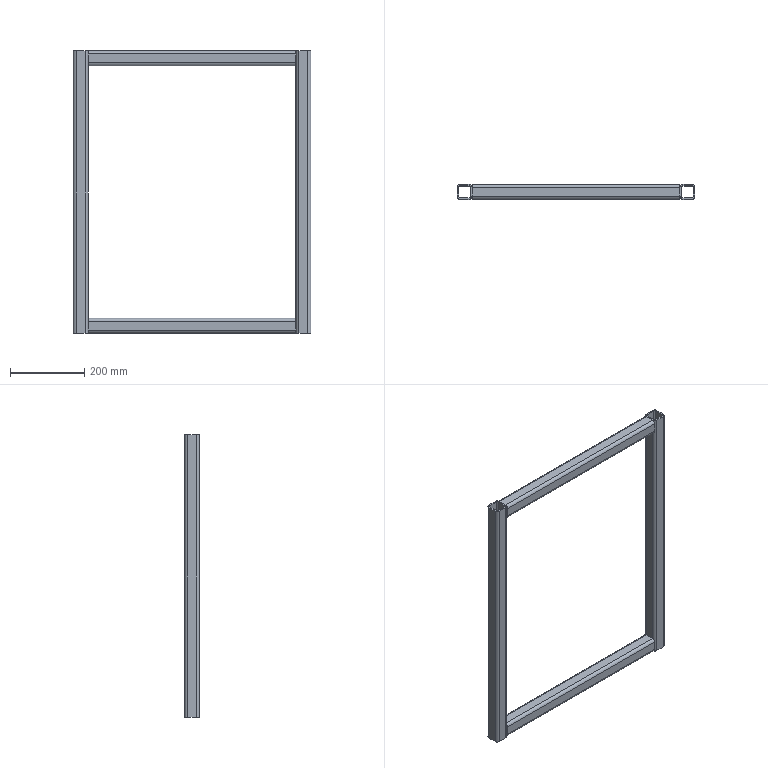Component | SolidWorks | 01-01Chassis-1_01-01-01ChassisWeldment1-1 | 4 solids | 74 faces | box 640 x 40 x 760 mm | volume 1411290 mm3 | plane 40 | cylinder 34 | commonest cylinder face diameters 8 x16 16 x16 13.5 x2 | material Q235
build123d program:
from build123d import *

# Parameters (mm, degrees)
SQUARE_TUBE_40_X_40_X_4_1_DEPTH   = 600
SQUARE_TUBE_40_X_40_X_4_1_2_DEPTH = 600
SQUARE_TUBE_40_X_40_X_4_2_DEPTH   = 720
SQUARE_TUBE_40_X_40_X_4_2_2_DEPTH = 720
BODY_3_RUN_ON_DEPTH               = 20
BODY_START                        = 720
BODY_3_RUN_ON_2_DEPTH             = 20
BODY_4_RUN_ON_DEPTH               = 20
BODY_4_RUN_ON_2_DEPTH             = 20
SKETCH13_R                        = 6.75
CUT_EXTRUDE1_DEPTH                = 10


with BuildPart() as part:
    # Sketch12 → Square Tube 40 X 40 X 4_1 (new body)
    with BuildSketch(Plane(origin=(300, 0, -360), x_dir=(0, 0, 1), z_dir=(-1, 0, 0))):
        with BuildLine():
            Line((-12, -20), (12, -20))
            ThreePointArc((12, -20), (17.657, -17.657), (20, -12))
            Line((20, -12), (20, 12))
            ThreePointArc((20, 12), (17.657, 17.657), (12, 20))
            Line((12, 20), (-12, 20))
            ThreePointArc((-12, 20), (-17.657, 17.657), (-20, 12))
            Line((-20, 12), (-20, -12))
            ThreePointArc((-20, -12), (-17.657, -17.657), (-12, -20))
        make_face()
        with BuildLine():
            Line((-12, -16), (12, -16))
            ThreePointArc((12, -16), (14.828, -14.828), (16, -12))
            Line((16, -12), (16, 12))
            ThreePointArc((16, 12), (14.828, 14.828), (12, 16))
            Line((12, 16), (-12, 16))
            ThreePointArc((-12, 16), (-14.828, 14.828), (-16, 12))
            Line((-16, 12), (-16, -12))
            ThreePointArc((-16, -12), (-14.828, -14.828), (-12, -16))
        make_face(mode=Mode.SUBTRACT)
    extrude(amount=SQUARE_TUBE_40_X_40_X_4_1_DEPTH)

    # Trim_Extend2 12
    split(bisect_by=Plane(origin=(-284, 0, 10), x_dir=(0, 1, 0), z_dir=(1, 0, 0)), keep=Keep.TOP)

    # Trim_Extend2 15
    split(bisect_by=Plane(origin=(-280, 0, 10), x_dir=(0, 1, 0), z_dir=(1, 0, 0)), keep=Keep.TOP)

    # Trim_Extend4 9
    split(bisect_by=Plane(origin=(280, 0, 0), x_dir=(0, -1, 0), z_dir=(-1, 0, 0)), keep=Keep.TOP)


with BuildPart() as body_2:
    # Sketch12 on segment 2 (on carried to segment 2) → Square Tube 40 X 40 X 4_1 2 (new body)
    with BuildSketch(Plane(origin=(300, 0, 360), x_dir=(0, 0, 1), z_dir=(-1, 0, 0))):
        with BuildLine():
            Line((-12, -20), (12, -20))
            ThreePointArc((12, -20), (17.657, -17.657), (20, -12))
            Line((20, -12), (20, 12))
            ThreePointArc((20, 12), (17.657, 17.657), (12, 20))
            Line((12, 20), (-12, 20))
            ThreePointArc((-12, 20), (-17.657, 17.657), (-20, 12))
            Line((-20, 12), (-20, -12))
            ThreePointArc((-20, -12), (-17.657, -17.657), (-12, -20))
        make_face()
        with BuildLine():
            Line((-12, -16), (12, -16))
            ThreePointArc((12, -16), (14.828, -14.828), (16, -12))
            Line((16, -12), (16, 12))
            ThreePointArc((16, 12), (14.828, 14.828), (12, 16))
            Line((12, 16), (-12, 16))
            ThreePointArc((-12, 16), (-14.828, 14.828), (-16, 12))
            Line((-16, 12), (-16, -12))
            ThreePointArc((-16, -12), (-14.828, -14.828), (-12, -16))
        make_face(mode=Mode.SUBTRACT)
    extrude(amount=SQUARE_TUBE_40_X_40_X_4_1_2_DEPTH)

    # Trim_Extend1 11
    split(bisect_by=Plane.YZ.offset(-280), keep=Keep.TOP)

    # Trim_Extend6 10
    split(bisect_by=Plane(origin=(284, 0, -10), x_dir=(0, -1, 0), z_dir=(-1, 0, 0)), keep=Keep.TOP)

    # Trim_Extend6 13
    split(bisect_by=Plane(origin=(280, 0, -10), x_dir=(0, -1, 0), z_dir=(-1, 0, 0)), keep=Keep.TOP)


with BuildPart() as body_3:
    # Sketch1 → Square Tube 40 X 40 X 4_2 (new body)
    with BuildSketch(Plane(origin=(-300, 0, 360), x_dir=(-1, 0, 0), z_dir=(0, 0, -1))):
        with BuildLine():
            Line((-12, -20), (12, -20))
            ThreePointArc((12, -20), (17.657, -17.657), (20, -12))
            Line((20, -12), (20, 12))
            ThreePointArc((20, 12), (17.657, 17.657), (12, 20))
            Line((12, 20), (-12, 20))
            ThreePointArc((-12, 20), (-17.657, 17.657), (-20, 12))
            Line((-20, 12), (-20, -12))
            ThreePointArc((-20, -12), (-17.657, -17.657), (-12, -20))
        make_face()
        with BuildLine():
            Line((-12, -16), (12, -16))
            ThreePointArc((12, -16), (14.828, -14.828), (16, -12))
            Line((16, -12), (16, 12))
            ThreePointArc((16, 12), (14.828, 14.828), (12, 16))
            Line((12, 16), (-12, 16))
            ThreePointArc((-12, 16), (-14.828, 14.828), (-16, 12))
            Line((-16, 12), (-16, -12))
            ThreePointArc((-16, -12), (-14.828, -14.828), (-12, -16))
        make_face(mode=Mode.SUBTRACT)
    extrude(amount=SQUARE_TUBE_40_X_40_X_4_2_DEPTH)

    # Sketch1 → body 3 run on (add)
    with BuildSketch(Plane(origin=(-300, 0, 360), x_dir=(-1, 0, 0), z_dir=(0, 0, -1))):
        with BuildLine():
            Line((-12, -20), (12, -20))
            ThreePointArc((12, -20), (17.657, -17.657), (20, -12))
            Line((20, -12), (20, 12))
            ThreePointArc((20, 12), (17.657, 17.657), (12, 20))
            Line((12, 20), (-12, 20))
            ThreePointArc((-12, 20), (-17.657, 17.657), (-20, 12))
            Line((-20, 12), (-20, -12))
            ThreePointArc((-20, -12), (-17.657, -17.657), (-12, -20))
        make_face()
        with BuildLine():
            Line((-12, -16), (12, -16))
            ThreePointArc((12, -16), (14.828, -14.828), (16, -12))
            Line((16, -12), (16, 12))
            ThreePointArc((16, 12), (14.828, 14.828), (12, 16))
            Line((12, 16), (-12, 16))
            ThreePointArc((-12, 16), (-14.828, 14.828), (-16, 12))
            Line((-16, 12), (-16, -12))
            ThreePointArc((-16, -12), (-14.828, -14.828), (-12, -16))
        make_face(mode=Mode.SUBTRACT)
    extrude(amount=-BODY_3_RUN_ON_DEPTH)

    # Sketch1 → body 3 run on 2 (add)
    with BuildSketch(Plane(origin=(-300, 0, 360), x_dir=(-1, 0, 0), z_dir=(0, 0, -1)).offset(BODY_START)):
        with BuildLine():
            Line((-12, -20), (12, -20))
            ThreePointArc((12, -20), (17.657, -17.657), (20, -12))
            Line((20, -12), (20, 12))
            ThreePointArc((20, 12), (17.657, 17.657), (12, 20))
            Line((12, 20), (-12, 20))
            ThreePointArc((-12, 20), (-17.657, 17.657), (-20, 12))
            Line((-20, 12), (-20, -12))
            ThreePointArc((-20, -12), (-17.657, -17.657), (-12, -20))
        make_face()
        with BuildLine():
            Line((-12, -16), (12, -16))
            ThreePointArc((12, -16), (14.828, -14.828), (16, -12))
            Line((16, -12), (16, 12))
            ThreePointArc((16, 12), (14.828, 14.828), (12, 16))
            Line((12, 16), (-12, 16))
            ThreePointArc((-12, 16), (-14.828, 14.828), (-16, 12))
            Line((-16, 12), (-16, -12))
            ThreePointArc((-16, -12), (-14.828, -14.828), (-12, -16))
        make_face(mode=Mode.SUBTRACT)
    extrude(amount=BODY_3_RUN_ON_2_DEPTH)


with BuildPart() as body_4:
    # Sketch1 on segment 2 (on carried to segment 2) → Square Tube 40 X 40 X 4_2 2 (new body)
    with BuildSketch(Plane(origin=(300, 0, 360), x_dir=(-1, 0, 0), z_dir=(0, 0, -1))):
        with BuildLine():
            Line((-12, -20), (12, -20))
            ThreePointArc((12, -20), (17.657, -17.657), (20, -12))
            Line((20, -12), (20, 12))
            ThreePointArc((20, 12), (17.657, 17.657), (12, 20))
            Line((12, 20), (-12, 20))
            ThreePointArc((-12, 20), (-17.657, 17.657), (-20, 12))
            Line((-20, 12), (-20, -12))
            ThreePointArc((-20, -12), (-17.657, -17.657), (-12, -20))
        make_face()
        with BuildLine():
            Line((-12, -16), (12, -16))
            ThreePointArc((12, -16), (14.828, -14.828), (16, -12))
            Line((16, -12), (16, 12))
            ThreePointArc((16, 12), (14.828, 14.828), (12, 16))
            Line((12, 16), (-12, 16))
            ThreePointArc((-12, 16), (-14.828, 14.828), (-16, 12))
            Line((-16, 12), (-16, -12))
            ThreePointArc((-16, -12), (-14.828, -14.828), (-12, -16))
        make_face(mode=Mode.SUBTRACT)
    extrude(amount=SQUARE_TUBE_40_X_40_X_4_2_2_DEPTH)

    # Sketch1 on segment 2 (on carried to segment 2) → body 4 run on (add)
    with BuildSketch(Plane(origin=(300, 0, 360), x_dir=(-1, 0, 0), z_dir=(0, 0, -1)).offset(BODY_START)):
        with BuildLine():
            Line((-12, -20), (12, -20))
            ThreePointArc((12, -20), (17.657, -17.657), (20, -12))
            Line((20, -12), (20, 12))
            ThreePointArc((20, 12), (17.657, 17.657), (12, 20))
            Line((12, 20), (-12, 20))
            ThreePointArc((-12, 20), (-17.657, 17.657), (-20, 12))
            Line((-20, 12), (-20, -12))
            ThreePointArc((-20, -12), (-17.657, -17.657), (-12, -20))
        make_face()
        with BuildLine():
            Line((-12, -16), (12, -16))
            ThreePointArc((12, -16), (14.828, -14.828), (16, -12))
            Line((16, -12), (16, 12))
            ThreePointArc((16, 12), (14.828, 14.828), (12, 16))
            Line((12, 16), (-12, 16))
            ThreePointArc((-12, 16), (-14.828, 14.828), (-16, 12))
            Line((-16, 12), (-16, -12))
            ThreePointArc((-16, -12), (-14.828, -14.828), (-12, -16))
        make_face(mode=Mode.SUBTRACT)
    extrude(amount=BODY_4_RUN_ON_DEPTH)

    # Sketch1 on segment 2 (on carried to segment 2) → body 4 run on 2 (add)
    with BuildSketch(Plane(origin=(300, 0, 360), x_dir=(-1, 0, 0), z_dir=(0, 0, -1))):
        with BuildLine():
            Line((-12, -20), (12, -20))
            ThreePointArc((12, -20), (17.657, -17.657), (20, -12))
            Line((20, -12), (20, 12))
            ThreePointArc((20, 12), (17.657, 17.657), (12, 20))
            Line((12, 20), (-12, 20))
            ThreePointArc((-12, 20), (-17.657, 17.657), (-20, 12))
            Line((-20, 12), (-20, -12))
            ThreePointArc((-20, -12), (-17.657, -17.657), (-12, -20))
        make_face()
        with BuildLine():
            Line((-12, -16), (12, -16))
            ThreePointArc((12, -16), (14.828, -14.828), (16, -12))
            Line((16, -12), (16, 12))
            ThreePointArc((16, 12), (14.828, 14.828), (12, 16))
            Line((12, 16), (-12, 16))
            ThreePointArc((-12, 16), (-14.828, 14.828), (-16, 12))
            Line((-16, 12), (-16, -12))
            ThreePointArc((-16, -12), (-14.828, -14.828), (-12, -16))
        make_face(mode=Mode.SUBTRACT)
    extrude(amount=-BODY_4_RUN_ON_2_DEPTH)

    # Sketch13 → Cut-Extrude1 (cut)
    with BuildSketch(Plane(origin=(0, 20, 0), x_dir=(1, 0, 0), z_dir=(0, 1, 0))):
        with Locations(Location((293.311, 32.684, 0), (0, 0, 218.107))):
            Circle(SKETCH13_R)
    extrude(amount=-CUT_EXTRUDE1_DEPTH, mode=Mode.SUBTRACT)


solid = Compound([part.part, body_2.part, body_3.part, body_4.part])

# Placed as in the assembly
solid = solid.moved(Location((0, 20, 0), (-180, 0, 180)))